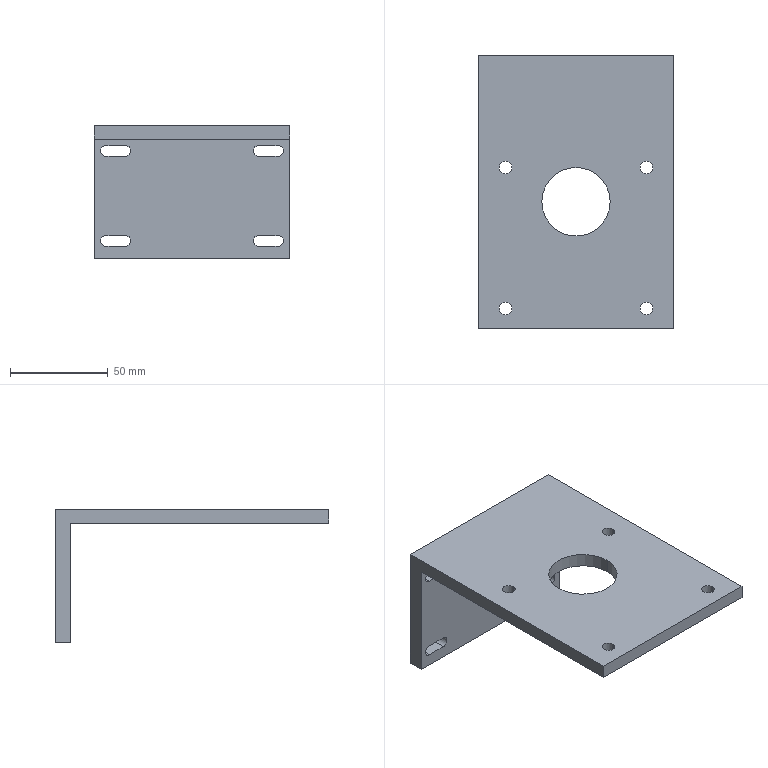Component | SolidWorks | --MA18S2004111xlMotorMountOutline2-1 | 1 solid | 34 faces | box 100 x 140 x 68 mm | volume 136616 mm3 | cylinder 18 | plane 16 | commonest cylinder face diameters 6.5 x8 5.5 x8 35 x2
STEP:
#1=CARTESIAN_POINT('',(11.226,-4.953,2.402));
#2=VERTEX_POINT('',#1);
#3=CARTESIAN_POINT('',(10.97,-4.953,2.402));
#4=VERTEX_POINT('',#3);
#5=CARTESIAN_POINT('',(11.098,-4.953,2.402));
#6=DIRECTION('',(0.,-0.,1.));
#7=DIRECTION('',(0.,-1.,0.));
#8=AXIS2_PLACEMENT_3D('',#5,#6,#7);
#9=CIRCLE('',#8,0.128);
#10=EDGE_CURVE('',#2,#4,#9,.T.);
#11=ORIENTED_EDGE('',*,*,#10,.F.);
#12=CARTESIAN_POINT('',(11.226,-4.953,2.677));
#13=VERTEX_POINT('',#12);
#14=CARTESIAN_POINT('',(11.226,-4.953,2.677));
#15=DIRECTION('',(0.,0.,1.));
#16=VECTOR('',#15,39.37);
#17=LINE('',#14,#16);
#18=EDGE_CURVE('',#2,#13,#17,.T.);
#19=ORIENTED_EDGE('',*,*,#18,.T.);
#20=CARTESIAN_POINT('',(10.97,-4.953,2.677));
#21=VERTEX_POINT('',#20);
#22=CARTESIAN_POINT('',(11.098,-4.953,2.677));
#23=DIRECTION('',(0.,0.,1.));
#24=DIRECTION('',(-1.,0.,0.));
#25=AXIS2_PLACEMENT_3D('',#22,#23,#24);
#26=CIRCLE('',#25,0.128);
#27=EDGE_CURVE('',#13,#21,#26,.T.);
#28=ORIENTED_EDGE('',*,*,#27,.T.);
#29=CARTESIAN_POINT('',(10.97,-4.953,2.677));
#30=DIRECTION('',(0.,0.,1.));
#31=VECTOR('',#30,39.37);
#32=LINE('',#29,#31);
#33=EDGE_CURVE('',#4,#21,#32,.T.);
#34=ORIENTED_EDGE('',*,*,#33,.F.);
#35=EDGE_LOOP('',(#11,#19,#28,#34));
#36=FACE_OUTER_BOUND('',#35,.T.);
#37=CARTESIAN_POINT('',(11.098,-4.953,2.677));
#38=DIRECTION('',(0.,0.,1.));
#39=DIRECTION('',(-1.,0.,0.));
#40=AXIS2_PLACEMENT_3D('',#37,#38,#39);
#41=CYLINDRICAL_SURFACE('',#40,0.128);
#42=ADVANCED_FACE('',(#36),#41,.F.);
#43=CARTESIAN_POINT('',(8.391,-4.953,2.402));
#44=VERTEX_POINT('',#43);
#45=CARTESIAN_POINT('',(8.135,-4.953,2.402));
#46=VERTEX_POINT('',#45);
#47=CARTESIAN_POINT('',(8.263,-4.953,2.402));
#48=DIRECTION('',(0.,-0.,1.));
#49=DIRECTION('',(0.,-1.,0.));
#50=AXIS2_PLACEMENT_3D('',#47,#48,#49);
#51=CIRCLE('',#50,0.128);
#52=EDGE_CURVE('',#44,#46,#51,.T.);
#53=ORIENTED_EDGE('',*,*,#52,.F.);
#54=CARTESIAN_POINT('',(8.391,-4.953,2.677));
#55=VERTEX_POINT('',#54);
#56=CARTESIAN_POINT('',(8.391,-4.953,2.677));
#57=DIRECTION('',(0.,0.,1.));
#58=VECTOR('',#57,39.37);
#59=LINE('',#56,#58);
#60=EDGE_CURVE('',#44,#55,#59,.T.);
#61=ORIENTED_EDGE('',*,*,#60,.T.);
#62=CARTESIAN_POINT('',(8.135,-4.953,2.677));
#63=VERTEX_POINT('',#62);
#64=CARTESIAN_POINT('',(8.263,-4.953,2.677));
#65=DIRECTION('',(0.,0.,1.));
#66=DIRECTION('',(-1.,0.,0.));
#67=AXIS2_PLACEMENT_3D('',#64,#65,#66);
#68=CIRCLE('',#67,0.128);
#69=EDGE_CURVE('',#55,#63,#68,.T.);
#70=ORIENTED_EDGE('',*,*,#69,.T.);
#71=CARTESIAN_POINT('',(8.135,-4.953,2.677));
#72=DIRECTION('',(0.,0.,1.));
#73=VECTOR('',#72,39.37);
#74=LINE('',#71,#73);
#75=EDGE_CURVE('',#46,#63,#74,.T.);
#76=ORIENTED_EDGE('',*,*,#75,.F.);
#77=EDGE_LOOP('',(#53,#61,#70,#76));
#78=FACE_OUTER_BOUND('',#77,.T.);
#79=CARTESIAN_POINT('',(8.263,-4.953,2.677));
#80=DIRECTION('',(0.,0.,1.));
#81=DIRECTION('',(-1.,0.,0.));
#82=AXIS2_PLACEMENT_3D('',#79,#80,#81);
#83=CYLINDRICAL_SURFACE('',#82,0.128);
#84=ADVANCED_FACE('',(#78),#83,.F.);
#85=CARTESIAN_POINT('',(11.226,-2.118,2.402));
#86=VERTEX_POINT('',#85);
#87=CARTESIAN_POINT('',(10.97,-2.118,2.402));
#88=VERTEX_POINT('',#87);
#89=CARTESIAN_POINT('',(11.098,-2.118,2.402));
#90=DIRECTION('',(0.,-0.,1.));
#91=DIRECTION('',(0.,-1.,0.));
#92=AXIS2_PLACEMENT_3D('',#89,#90,#91);
#93=CIRCLE('',#92,0.128);
#94=EDGE_CURVE('',#86,#88,#93,.T.);
#95=ORIENTED_EDGE('',*,*,#94,.F.);
#96=CARTESIAN_POINT('',(11.226,-2.118,2.677));
#97=VERTEX_POINT('',#96);
#98=CARTESIAN_POINT('',(11.226,-2.118,2.677));
#99=DIRECTION('',(0.,0.,1.));
#100=VECTOR('',#99,39.37);
#101=LINE('',#98,#100);
#102=EDGE_CURVE('',#86,#97,#101,.T.);
#103=ORIENTED_EDGE('',*,*,#102,.T.);
#104=CARTESIAN_POINT('',(10.97,-2.118,2.677));
#105=VERTEX_POINT('',#104);
#106=CARTESIAN_POINT('',(11.098,-2.118,2.677));
#107=DIRECTION('',(0.,0.,1.));
#108=DIRECTION('',(-1.,0.,0.));
#109=AXIS2_PLACEMENT_3D('',#106,#107,#108);
#110=CIRCLE('',#109,0.128);
#111=EDGE_CURVE('',#97,#105,#110,.T.);
#112=ORIENTED_EDGE('',*,*,#111,.T.);
#113=CARTESIAN_POINT('',(10.97,-2.118,2.677));
#114=DIRECTION('',(0.,0.,1.));
#115=VECTOR('',#114,39.37);
#116=LINE('',#113,#115);
#117=EDGE_CURVE('',#88,#105,#116,.T.);
#118=ORIENTED_EDGE('',*,*,#117,.F.);
#119=EDGE_LOOP('',(#95,#103,#112,#118));
#120=FACE_OUTER_BOUND('',#119,.T.);
#121=CARTESIAN_POINT('',(11.098,-2.118,2.677));
#122=DIRECTION('',(0.,0.,1.));
#123=DIRECTION('',(-1.,0.,0.));
#124=AXIS2_PLACEMENT_3D('',#121,#122,#123);
#125=CYLINDRICAL_SURFACE('',#124,0.128);
#126=ADVANCED_FACE('',(#120),#125,.F.);
#127=CARTESIAN_POINT('',(8.391,-2.118,2.402));
#128=VERTEX_POINT('',#127);
#129=CARTESIAN_POINT('',(8.135,-2.118,2.402));
#130=VERTEX_POINT('',#129);
#131=CARTESIAN_POINT('',(8.263,-2.118,2.402));
#132=DIRECTION('',(0.,-0.,1.));
#133=DIRECTION('',(0.,-1.,0.));
#134=AXIS2_PLACEMENT_3D('',#131,#132,#133);
#135=CIRCLE('',#134,0.128);
#136=EDGE_CURVE('',#128,#130,#135,.T.);
#137=ORIENTED_EDGE('',*,*,#136,.F.);
#138=CARTESIAN_POINT('',(8.391,-2.118,2.677));
#139=VERTEX_POINT('',#138);
#140=CARTESIAN_POINT('',(8.391,-2.118,2.677));
#141=DIRECTION('',(0.,0.,1.));
#142=VECTOR('',#141,39.37);
#143=LINE('',#140,#142);
#144=EDGE_CURVE('',#128,#139,#143,.T.);
#145=ORIENTED_EDGE('',*,*,#144,.T.);
#146=CARTESIAN_POINT('',(8.135,-2.118,2.677));
#147=VERTEX_POINT('',#146);
#148=CARTESIAN_POINT('',(8.263,-2.118,2.677));
#149=DIRECTION('',(0.,0.,1.));
#150=DIRECTION('',(-1.,0.,0.));
#151=AXIS2_PLACEMENT_3D('',#148,#149,#150);
#152=CIRCLE('',#151,0.128);
#153=EDGE_CURVE('',#139,#147,#152,.T.);
#154=ORIENTED_EDGE('',*,*,#153,.T.);
#155=CARTESIAN_POINT('',(8.135,-2.118,2.677));
#156=DIRECTION('',(0.,0.,1.));
#157=VECTOR('',#156,39.37);
#158=LINE('',#155,#157);
#159=EDGE_CURVE('',#130,#147,#158,.T.);
#160=ORIENTED_EDGE('',*,*,#159,.F.);
#161=EDGE_LOOP('',(#137,#145,#154,#160));
#162=FACE_OUTER_BOUND('',#161,.T.);
#163=CARTESIAN_POINT('',(8.263,-2.118,2.677));
#164=DIRECTION('',(0.,0.,1.));
#165=DIRECTION('',(-1.,0.,0.));
#166=AXIS2_PLACEMENT_3D('',#163,#164,#165);
#167=CYLINDRICAL_SURFACE('',#166,0.128);
#168=ADVANCED_FACE('',(#162),#167,.F.);
#169=CARTESIAN_POINT('',(10.369,-2.807,2.402));
#170=VERTEX_POINT('',#169);
#171=CARTESIAN_POINT('',(8.992,-2.807,2.402));
#172=VERTEX_POINT('',#171);
#173=CARTESIAN_POINT('',(9.681,-2.807,2.402));
#174=DIRECTION('',(0.,-0.,1.));
#175=DIRECTION('',(0.,-1.,0.));
#176=AXIS2_PLACEMENT_3D('',#173,#174,#175);
#177=CIRCLE('',#176,0.689);
#178=EDGE_CURVE('',#170,#172,#177,.T.);
#179=ORIENTED_EDGE('',*,*,#178,.F.);
#180=CARTESIAN_POINT('',(10.369,-2.807,2.677));
#181=VERTEX_POINT('',#180);
#182=CARTESIAN_POINT('',(10.369,-2.807,0.));
#183=DIRECTION('',(0.,0.,1.));
#184=VECTOR('',#183,39.37);
#185=LINE('',#182,#184);
#186=EDGE_CURVE('',#170,#181,#185,.T.);
#187=ORIENTED_EDGE('',*,*,#186,.T.);
#188=CARTESIAN_POINT('',(8.992,-2.807,2.677));
#189=VERTEX_POINT('',#188);
#190=CARTESIAN_POINT('',(9.681,-2.807,2.677));
#191=DIRECTION('',(0.,0.,1.));
#192=DIRECTION('',(-1.,0.,0.));
#193=AXIS2_PLACEMENT_3D('',#190,#191,#192);
#194=CIRCLE('',#193,0.689);
#195=EDGE_CURVE('',#181,#189,#194,.T.);
#196=ORIENTED_EDGE('',*,*,#195,.T.);
#197=CARTESIAN_POINT('',(8.992,-2.807,0.));
#198=DIRECTION('',(0.,0.,1.));
#199=VECTOR('',#198,39.37);
#200=LINE('',#197,#199);
#201=EDGE_CURVE('',#172,#189,#200,.T.);
#202=ORIENTED_EDGE('',*,*,#201,.F.);
#203=EDGE_LOOP('',(#179,#187,#196,#202));
#204=FACE_OUTER_BOUND('',#203,.T.);
#205=CARTESIAN_POINT('',(9.681,-2.807,0.));
#206=DIRECTION('',(0.,0.,1.));
#207=DIRECTION('',(-1.,0.,0.));
#208=AXIS2_PLACEMENT_3D('',#205,#206,#207);
#209=CYLINDRICAL_SURFACE('',#208,0.689);
#210=ADVANCED_FACE('',(#204),#209,.F.);
#211=CARTESIAN_POINT('',(7.948,0.1456,2.057));
#212=VERTEX_POINT('',#211);
#213=CARTESIAN_POINT('',(8.342,0.1456,2.057));
#214=VERTEX_POINT('',#213);
#215=CARTESIAN_POINT('',(8.342,0.1456,2.057));
#216=DIRECTION('',(1.,0.,0.));
#217=VECTOR('',#216,39.37);
#218=LINE('',#215,#217);
#219=EDGE_CURVE('',#212,#214,#218,.T.);
#220=ORIENTED_EDGE('',*,*,#219,.T.);
#221=CARTESIAN_POINT('',(8.342,0.1456,2.274));
#222=VERTEX_POINT('',#221);
#223=CARTESIAN_POINT('',(8.342,0.1456,2.165));
#224=DIRECTION('',(0.,-1.,-0.));
#225=DIRECTION('',(0.,0.,-1.));
#226=AXIS2_PLACEMENT_3D('',#223,#224,#225);
#227=CIRCLE('',#226,0.1083);
#228=EDGE_CURVE('',#214,#222,#227,.T.);
#229=ORIENTED_EDGE('',*,*,#228,.T.);
#230=CARTESIAN_POINT('',(7.948,0.1456,2.274));
#231=VERTEX_POINT('',#230);
#232=CARTESIAN_POINT('',(8.342,0.1456,2.274));
#233=DIRECTION('',(-1.,0.,0.));
#234=VECTOR('',#233,39.37);
#235=LINE('',#232,#234);
#236=EDGE_CURVE('',#222,#231,#235,.T.);
#237=ORIENTED_EDGE('',*,*,#236,.T.);
#238=CARTESIAN_POINT('',(7.948,0.1456,2.165));
#239=DIRECTION('',(0.,-1.,-0.));
#240=DIRECTION('',(0.,0.,-1.));
#241=AXIS2_PLACEMENT_3D('',#238,#239,#240);
#242=CIRCLE('',#241,0.1083);
#243=EDGE_CURVE('',#231,#212,#242,.T.);
#244=ORIENTED_EDGE('',*,*,#243,.T.);
#245=EDGE_LOOP('',(#220,#229,#237,#244));
#246=FACE_BOUND('',#245,.T.);
#247=CARTESIAN_POINT('',(11.019,0.1456,2.057));
#248=VERTEX_POINT('',#247);
#249=CARTESIAN_POINT('',(11.413,0.1456,2.057));
#250=VERTEX_POINT('',#249);
#251=CARTESIAN_POINT('',(11.413,0.1456,2.057));
#252=DIRECTION('',(1.,0.,0.));
#253=VECTOR('',#252,39.37);
#254=LINE('',#251,#253);
#255=EDGE_CURVE('',#248,#250,#254,.T.);
#256=ORIENTED_EDGE('',*,*,#255,.T.);
#257=CARTESIAN_POINT('',(11.413,0.1456,2.274));
#258=VERTEX_POINT('',#257);
#259=CARTESIAN_POINT('',(11.413,0.1456,2.165));
#260=DIRECTION('',(0.,-1.,-0.));
#261=DIRECTION('',(0.,0.,-1.));
#262=AXIS2_PLACEMENT_3D('',#259,#260,#261);
#263=CIRCLE('',#262,0.1083);
#264=EDGE_CURVE('',#250,#258,#263,.T.);
#265=ORIENTED_EDGE('',*,*,#264,.T.);
#266=CARTESIAN_POINT('',(11.019,0.1456,2.274));
#267=VERTEX_POINT('',#266);
#268=CARTESIAN_POINT('',(11.413,0.1456,2.274));
#269=DIRECTION('',(-1.,0.,0.));
#270=VECTOR('',#269,39.37);
#271=LINE('',#268,#270);
#272=EDGE_CURVE('',#258,#267,#271,.T.);
#273=ORIENTED_EDGE('',*,*,#272,.T.);
#274=CARTESIAN_POINT('',(11.019,0.1456,2.165));
#275=DIRECTION('',(0.,-1.,-0.));
#276=DIRECTION('',(0.,0.,-1.));
#277=AXIS2_PLACEMENT_3D('',#274,#275,#276);
#278=CIRCLE('',#277,0.1083);
#279=EDGE_CURVE('',#267,#248,#278,.T.);
#280=ORIENTED_EDGE('',*,*,#279,.T.);
#281=EDGE_LOOP('',(#256,#265,#273,#280));
#282=FACE_BOUND('',#281,.T.);
#283=CARTESIAN_POINT('',(7.948,0.1456,0.2461));
#284=VERTEX_POINT('',#283);
#285=CARTESIAN_POINT('',(8.342,0.1456,0.2461));
#286=VERTEX_POINT('',#285);
#287=CARTESIAN_POINT('',(8.342,0.1456,0.2461));
#288=DIRECTION('',(1.,0.,0.));
#289=VECTOR('',#288,39.37);
#290=LINE('',#287,#289);
#291=EDGE_CURVE('',#284,#286,#290,.T.);
#292=ORIENTED_EDGE('',*,*,#291,.T.);
#293=CARTESIAN_POINT('',(8.342,0.1456,0.4626));
#294=VERTEX_POINT('',#293);
#295=CARTESIAN_POINT('',(8.342,0.1456,0.3543));
#296=DIRECTION('',(0.,-1.,-0.));
#297=DIRECTION('',(0.,0.,-1.));
#298=AXIS2_PLACEMENT_3D('',#295,#296,#297);
#299=CIRCLE('',#298,0.1083);
#300=EDGE_CURVE('',#286,#294,#299,.T.);
#301=ORIENTED_EDGE('',*,*,#300,.T.);
#302=CARTESIAN_POINT('',(7.948,0.1456,0.4626));
#303=VERTEX_POINT('',#302);
#304=CARTESIAN_POINT('',(8.342,0.1456,0.4626));
#305=DIRECTION('',(-1.,0.,0.));
#306=VECTOR('',#305,39.37);
#307=LINE('',#304,#306);
#308=EDGE_CURVE('',#294,#303,#307,.T.);
#309=ORIENTED_EDGE('',*,*,#308,.T.);
#310=CARTESIAN_POINT('',(7.948,0.1456,0.3543));
#311=DIRECTION('',(0.,-1.,-0.));
#312=DIRECTION('',(0.,0.,-1.));
#313=AXIS2_PLACEMENT_3D('',#310,#311,#312);
#314=CIRCLE('',#313,0.1083);
#315=EDGE_CURVE('',#303,#284,#314,.T.);
#316=ORIENTED_EDGE('',*,*,#315,.T.);
#317=EDGE_LOOP('',(#292,#301,#309,#316));
#318=FACE_BOUND('',#317,.T.);
#319=CARTESIAN_POINT('',(11.019,0.1456,0.2461));
#320=VERTEX_POINT('',#319);
#321=CARTESIAN_POINT('',(11.413,0.1456,0.2461));
#322=VERTEX_POINT('',#321);
#323=CARTESIAN_POINT('',(11.413,0.1456,0.2461));
#324=DIRECTION('',(1.,0.,0.));
#325=VECTOR('',#324,39.37);
#326=LINE('',#323,#325);
#327=EDGE_CURVE('',#320,#322,#326,.T.);
#328=ORIENTED_EDGE('',*,*,#327,.T.);
#329=CARTESIAN_POINT('',(11.413,0.1456,0.4626));
#330=VERTEX_POINT('',#329);
#331=CARTESIAN_POINT('',(11.413,0.1456,0.3543));
#332=DIRECTION('',(0.,-1.,-0.));
#333=DIRECTION('',(0.,0.,-1.));
#334=AXIS2_PLACEMENT_3D('',#331,#332,#333);
#335=CIRCLE('',#334,0.1083);
#336=EDGE_CURVE('',#322,#330,#335,.T.);
#337=ORIENTED_EDGE('',*,*,#336,.T.);
#338=CARTESIAN_POINT('',(11.019,0.1456,0.4626));
#339=VERTEX_POINT('',#338);
#340=CARTESIAN_POINT('',(11.413,0.1456,0.4626));
#341=DIRECTION('',(-1.,0.,0.));
#342=VECTOR('',#341,39.37);
#343=LINE('',#340,#342);
#344=EDGE_CURVE('',#330,#339,#343,.T.);
#345=ORIENTED_EDGE('',*,*,#344,.T.);
#346=CARTESIAN_POINT('',(11.019,0.1456,0.3543));
#347=DIRECTION('',(0.,-1.,-0.));
#348=DIRECTION('',(0.,0.,-1.));
#349=AXIS2_PLACEMENT_3D('',#346,#347,#348);
#350=CIRCLE('',#349,0.1083);
#351=EDGE_CURVE('',#339,#320,#350,.T.);
#352=ORIENTED_EDGE('',*,*,#351,.T.);
#353=EDGE_LOOP('',(#328,#337,#345,#352));
#354=FACE_BOUND('',#353,.T.);
#355=CARTESIAN_POINT('',(7.712,0.1456,0.));
#356=VERTEX_POINT('',#355);
#357=CARTESIAN_POINT('',(7.712,0.1456,2.677));
#358=VERTEX_POINT('',#357);
#359=CARTESIAN_POINT('',(7.712,0.1456,2.677));
#360=DIRECTION('',(0.,0.,1.));
#361=VECTOR('',#360,39.37);
#362=LINE('',#359,#361);
#363=EDGE_CURVE('',#356,#358,#362,.T.);
#364=ORIENTED_EDGE('',*,*,#363,.T.);
#365=CARTESIAN_POINT('',(11.649,0.1456,2.677));
#366=VERTEX_POINT('',#365);
#367=CARTESIAN_POINT('',(11.649,0.1456,2.677));
#368=DIRECTION('',(-1.,0.,0.));
#369=VECTOR('',#368,39.37);
#370=LINE('',#367,#369);
#371=EDGE_CURVE('',#366,#358,#370,.T.);
#372=ORIENTED_EDGE('',*,*,#371,.F.);
#373=CARTESIAN_POINT('',(11.649,0.1456,0.));
#374=VERTEX_POINT('',#373);
#375=CARTESIAN_POINT('',(11.649,0.1456,2.677));
#376=DIRECTION('',(0.,0.,1.));
#377=VECTOR('',#376,39.37);
#378=LINE('',#375,#377);
#379=EDGE_CURVE('',#374,#366,#378,.T.);
#380=ORIENTED_EDGE('',*,*,#379,.F.);
#381=CARTESIAN_POINT('',(11.649,0.1456,0.));
#382=DIRECTION('',(-1.,0.,0.));
#383=VECTOR('',#382,39.37);
#384=LINE('',#381,#383);
#385=EDGE_CURVE('',#374,#356,#384,.T.);
#386=ORIENTED_EDGE('',*,*,#385,.T.);
#387=EDGE_LOOP('',(#364,#372,#380,#386));
#388=FACE_OUTER_BOUND('',#387,.T.);
#389=CARTESIAN_POINT('',(11.649,0.1456,2.677));
#390=DIRECTION('',(0.,-1.,0.));
#391=DIRECTION('',(-1.,0.,0.));
#392=AXIS2_PLACEMENT_3D('',#389,#390,#391);
#393=PLANE('',#392);
#394=ADVANCED_FACE('',(#246,#282,#318,#354,#388),#393,.F.);
#395=CARTESIAN_POINT('',(11.098,-4.953,2.677));
#396=DIRECTION('',(0.,0.,1.));
#397=DIRECTION('',(-1.,0.,0.));
#398=AXIS2_PLACEMENT_3D('',#395,#396,#397);
#399=CIRCLE('',#398,0.128);
#400=EDGE_CURVE('',#21,#13,#399,.T.);
#401=ORIENTED_EDGE('',*,*,#400,.F.);
#402=ORIENTED_EDGE('',*,*,#27,.F.);
#403=EDGE_LOOP('',(#401,#402));
#404=FACE_BOUND('',#403,.T.);
#405=CARTESIAN_POINT('',(8.263,-4.953,2.677));
#406=DIRECTION('',(0.,0.,1.));
#407=DIRECTION('',(-1.,0.,0.));
#408=AXIS2_PLACEMENT_3D('',#405,#406,#407);
#409=CIRCLE('',#408,0.128);
#410=EDGE_CURVE('',#63,#55,#409,.T.);
#411=ORIENTED_EDGE('',*,*,#410,.F.);
#412=ORIENTED_EDGE('',*,*,#69,.F.);
#413=EDGE_LOOP('',(#411,#412));
#414=FACE_BOUND('',#413,.T.);
#415=CARTESIAN_POINT('',(11.098,-2.118,2.677));
#416=DIRECTION('',(0.,0.,1.));
#417=DIRECTION('',(-1.,0.,0.));
#418=AXIS2_PLACEMENT_3D('',#415,#416,#417);
#419=CIRCLE('',#418,0.128);
#420=EDGE_CURVE('',#105,#97,#419,.T.);
#421=ORIENTED_EDGE('',*,*,#420,.F.);
#422=ORIENTED_EDGE('',*,*,#111,.F.);
#423=EDGE_LOOP('',(#421,#422));
#424=FACE_BOUND('',#423,.T.);
#425=CARTESIAN_POINT('',(8.263,-2.118,2.677));
#426=DIRECTION('',(0.,0.,1.));
#427=DIRECTION('',(-1.,0.,0.));
#428=AXIS2_PLACEMENT_3D('',#425,#426,#427);
#429=CIRCLE('',#428,0.128);
#430=EDGE_CURVE('',#147,#139,#429,.T.);
#431=ORIENTED_EDGE('',*,*,#430,.F.);
#432=ORIENTED_EDGE('',*,*,#153,.F.);
#433=EDGE_LOOP('',(#431,#432));
#434=FACE_BOUND('',#433,.T.);
#435=CARTESIAN_POINT('',(9.681,-2.807,2.677));
#436=DIRECTION('',(0.,0.,1.));
#437=DIRECTION('',(-1.,0.,0.));
#438=AXIS2_PLACEMENT_3D('',#435,#436,#437);
#439=CIRCLE('',#438,0.689);
#440=EDGE_CURVE('',#189,#181,#439,.T.);
#441=ORIENTED_EDGE('',*,*,#440,.F.);
#442=ORIENTED_EDGE('',*,*,#195,.F.);
#443=EDGE_LOOP('',(#441,#442));
#444=FACE_BOUND('',#443,.T.);
#445=CARTESIAN_POINT('',(7.712,-5.366,2.677));
#446=VERTEX_POINT('',#445);
#447=CARTESIAN_POINT('',(7.712,0.1456,2.677));
#448=DIRECTION('',(0.,-1.,0.));
#449=VECTOR('',#448,39.37);
#450=LINE('',#447,#449);
#451=EDGE_CURVE('',#358,#446,#450,.T.);
#452=ORIENTED_EDGE('',*,*,#451,.T.);
#453=CARTESIAN_POINT('',(11.649,-5.366,2.677));
#454=VERTEX_POINT('',#453);
#455=CARTESIAN_POINT('',(11.649,-5.366,2.677));
#456=DIRECTION('',(-1.,0.,0.));
#457=VECTOR('',#456,39.37);
#458=LINE('',#455,#457);
#459=EDGE_CURVE('',#454,#446,#458,.T.);
#460=ORIENTED_EDGE('',*,*,#459,.F.);
#461=CARTESIAN_POINT('',(11.649,0.1456,2.677));
#462=DIRECTION('',(0.,-1.,0.));
#463=VECTOR('',#462,39.37);
#464=LINE('',#461,#463);
#465=EDGE_CURVE('',#366,#454,#464,.T.);
#466=ORIENTED_EDGE('',*,*,#465,.F.);
#467=ORIENTED_EDGE('',*,*,#371,.T.);
#468=EDGE_LOOP('',(#452,#460,#466,#467));
#469=FACE_OUTER_BOUND('',#468,.T.);
#470=CARTESIAN_POINT('',(11.649,0.1456,2.677));
#471=DIRECTION('',(0.,0.,-1.));
#472=DIRECTION('',(1.,0.,0.));
#473=AXIS2_PLACEMENT_3D('',#470,#471,#472);
#474=PLANE('',#473);
#475=ADVANCED_FACE('',(#404,#414,#424,#434,#444,#469),#474,.F.);
#476=CARTESIAN_POINT('',(7.712,-5.366,2.402));
#477=VERTEX_POINT('',#476);
#478=CARTESIAN_POINT('',(7.712,-5.366,2.677));
#479=DIRECTION('',(0.,0.,-1.));
#480=VECTOR('',#479,39.37);
#481=LINE('',#478,#480);
#482=EDGE_CURVE('',#446,#477,#481,.T.);
#483=ORIENTED_EDGE('',*,*,#482,.T.);
#484=CARTESIAN_POINT('',(11.649,-5.366,2.402));
#485=VERTEX_POINT('',#484);
#486=CARTESIAN_POINT('',(11.649,-5.366,2.402));
#487=DIRECTION('',(-1.,0.,0.));
#488=VECTOR('',#487,39.37);
#489=LINE('',#486,#488);
#490=EDGE_CURVE('',#485,#477,#489,.T.);
#491=ORIENTED_EDGE('',*,*,#490,.F.);
#492=CARTESIAN_POINT('',(11.649,-5.366,2.677));
#493=DIRECTION('',(0.,0.,-1.));
#494=VECTOR('',#493,39.37);
#495=LINE('',#492,#494);
#496=EDGE_CURVE('',#454,#485,#495,.T.);
#497=ORIENTED_EDGE('',*,*,#496,.F.);
#498=ORIENTED_EDGE('',*,*,#459,.T.);
#499=EDGE_LOOP('',(#483,#491,#497,#498));
#500=FACE_OUTER_BOUND('',#499,.T.);
#501=CARTESIAN_POINT('',(11.649,-5.366,2.677));
#502=DIRECTION('',(0.,1.,0.));
#503=DIRECTION('',(1.,0.,0.));
#504=AXIS2_PLACEMENT_3D('',#501,#502,#503);
#505=PLANE('',#504);
#506=ADVANCED_FACE('',(#500),#505,.F.);
#507=CARTESIAN_POINT('',(11.098,-4.953,2.402));
#508=DIRECTION('',(0.,-0.,1.));
#509=DIRECTION('',(0.,-1.,0.));
#510=AXIS2_PLACEMENT_3D('',#507,#508,#509);
#511=CIRCLE('',#510,0.128);
#512=EDGE_CURVE('',#4,#2,#511,.T.);
#513=ORIENTED_EDGE('',*,*,#512,.T.);
#514=ORIENTED_EDGE('',*,*,#10,.T.);
#515=EDGE_LOOP('',(#513,#514));
#516=FACE_BOUND('',#515,.T.);
#517=CARTESIAN_POINT('',(8.263,-4.953,2.402));
#518=DIRECTION('',(0.,-0.,1.));
#519=DIRECTION('',(0.,-1.,0.));
#520=AXIS2_PLACEMENT_3D('',#517,#518,#519);
#521=CIRCLE('',#520,0.128);
#522=EDGE_CURVE('',#46,#44,#521,.T.);
#523=ORIENTED_EDGE('',*,*,#522,.T.);
#524=ORIENTED_EDGE('',*,*,#52,.T.);
#525=EDGE_LOOP('',(#523,#524));
#526=FACE_BOUND('',#525,.T.);
#527=CARTESIAN_POINT('',(11.098,-2.118,2.402));
#528=DIRECTION('',(0.,-0.,1.));
#529=DIRECTION('',(0.,-1.,0.));
#530=AXIS2_PLACEMENT_3D('',#527,#528,#529);
#531=CIRCLE('',#530,0.128);
#532=EDGE_CURVE('',#88,#86,#531,.T.);
#533=ORIENTED_EDGE('',*,*,#532,.T.);
#534=ORIENTED_EDGE('',*,*,#94,.T.);
#535=EDGE_LOOP('',(#533,#534));
#536=FACE_BOUND('',#535,.T.);
#537=CARTESIAN_POINT('',(8.263,-2.118,2.402));
#538=DIRECTION('',(0.,-0.,1.));
#539=DIRECTION('',(0.,-1.,0.));
#540=AXIS2_PLACEMENT_3D('',#537,#538,#539);
#541=CIRCLE('',#540,0.128);
#542=EDGE_CURVE('',#130,#128,#541,.T.);
#543=ORIENTED_EDGE('',*,*,#542,.T.);
#544=ORIENTED_EDGE('',*,*,#136,.T.);
#545=EDGE_LOOP('',(#543,#544));
#546=FACE_BOUND('',#545,.T.);
#547=CARTESIAN_POINT('',(9.681,-2.807,2.402));
#548=DIRECTION('',(0.,-0.,1.));
#549=DIRECTION('',(0.,-1.,0.));
#550=AXIS2_PLACEMENT_3D('',#547,#548,#549);
#551=CIRCLE('',#550,0.689);
#552=EDGE_CURVE('',#172,#170,#551,.T.);
#553=ORIENTED_EDGE('',*,*,#552,.T.);
#554=ORIENTED_EDGE('',*,*,#178,.T.);
#555=EDGE_LOOP('',(#553,#554));
#556=FACE_BOUND('',#555,.T.);
#557=CARTESIAN_POINT('',(7.712,-0.1693,2.402));
#558=VERTEX_POINT('',#557);
#559=CARTESIAN_POINT('',(7.712,-5.366,2.402));
#560=DIRECTION('',(0.,1.,0.));
#561=VECTOR('',#560,39.37);
#562=LINE('',#559,#561);
#563=EDGE_CURVE('',#477,#558,#562,.T.);
#564=ORIENTED_EDGE('',*,*,#563,.T.);
#565=CARTESIAN_POINT('',(11.649,-0.1693,2.402));
#566=VERTEX_POINT('',#565);
#567=CARTESIAN_POINT('',(11.649,-0.1693,2.402));
#568=DIRECTION('',(-1.,0.,0.));
#569=VECTOR('',#568,39.37);
#570=LINE('',#567,#569);
#571=EDGE_CURVE('',#566,#558,#570,.T.);
#572=ORIENTED_EDGE('',*,*,#571,.F.);
#573=CARTESIAN_POINT('',(11.649,-5.366,2.402));
#574=DIRECTION('',(0.,1.,0.));
#575=VECTOR('',#574,39.37);
#576=LINE('',#573,#575);
#577=EDGE_CURVE('',#485,#566,#576,.T.);
#578=ORIENTED_EDGE('',*,*,#577,.F.);
#579=ORIENTED_EDGE('',*,*,#490,.T.);
#580=EDGE_LOOP('',(#564,#572,#578,#579));
#581=FACE_OUTER_BOUND('',#580,.T.);
#582=CARTESIAN_POINT('',(11.649,-5.366,2.402));
#583=DIRECTION('',(0.,-0.,1.));
#584=DIRECTION('',(0.,-1.,-0.));
#585=AXIS2_PLACEMENT_3D('',#582,#583,#584);
#586=PLANE('',#585);
#587=ADVANCED_FACE('',(#516,#526,#536,#546,#556,#581),#586,.F.);
#588=CARTESIAN_POINT('',(8.342,-0.1693,2.274));
#589=VERTEX_POINT('',#588);
#590=CARTESIAN_POINT('',(7.948,-0.1693,2.274));
#591=VERTEX_POINT('',#590);
#592=CARTESIAN_POINT('',(8.342,-0.1693,2.274));
#593=DIRECTION('',(-1.,0.,0.));
#594=VECTOR('',#593,39.37);
#595=LINE('',#592,#594);
#596=EDGE_CURVE('',#589,#591,#595,.T.);
#597=ORIENTED_EDGE('',*,*,#596,.F.);
#598=CARTESIAN_POINT('',(8.342,-0.1693,2.057));
#599=VERTEX_POINT('',#598);
#600=CARTESIAN_POINT('',(8.342,-0.1693,2.165));
#601=DIRECTION('',(0.,-1.,-0.));
#602=DIRECTION('',(0.,0.,-1.));
#603=AXIS2_PLACEMENT_3D('',#600,#601,#602);
#604=CIRCLE('',#603,0.1083);
#605=EDGE_CURVE('',#599,#589,#604,.T.);
#606=ORIENTED_EDGE('',*,*,#605,.F.);
#607=CARTESIAN_POINT('',(7.948,-0.1693,2.057));
#608=VERTEX_POINT('',#607);
#609=CARTESIAN_POINT('',(8.342,-0.1693,2.057));
#610=DIRECTION('',(1.,0.,0.));
#611=VECTOR('',#610,39.37);
#612=LINE('',#609,#611);
#613=EDGE_CURVE('',#608,#599,#612,.T.);
#614=ORIENTED_EDGE('',*,*,#613,.F.);
#615=CARTESIAN_POINT('',(7.948,-0.1693,2.165));
#616=DIRECTION('',(0.,-1.,-0.));
#617=DIRECTION('',(0.,0.,-1.));
#618=AXIS2_PLACEMENT_3D('',#615,#616,#617);
#619=CIRCLE('',#618,0.1083);
#620=EDGE_CURVE('',#591,#608,#619,.T.);
#621=ORIENTED_EDGE('',*,*,#620,.F.);
#622=EDGE_LOOP('',(#597,#606,#614,#621));
#623=FACE_BOUND('',#622,.T.);
#624=CARTESIAN_POINT('',(11.413,-0.1693,2.274));
#625=VERTEX_POINT('',#624);
#626=CARTESIAN_POINT('',(11.019,-0.1693,2.274));
#627=VERTEX_POINT('',#626);
#628=CARTESIAN_POINT('',(11.413,-0.1693,2.274));
#629=DIRECTION('',(-1.,0.,0.));
#630=VECTOR('',#629,39.37);
#631=LINE('',#628,#630);
#632=EDGE_CURVE('',#625,#627,#631,.T.);
#633=ORIENTED_EDGE('',*,*,#632,.F.);
#634=CARTESIAN_POINT('',(11.413,-0.1693,2.057));
#635=VERTEX_POINT('',#634);
#636=CARTESIAN_POINT('',(11.413,-0.1693,2.165));
#637=DIRECTION('',(0.,-1.,-0.));
#638=DIRECTION('',(0.,0.,-1.));
#639=AXIS2_PLACEMENT_3D('',#636,#637,#638);
#640=CIRCLE('',#639,0.1083);
#641=EDGE_CURVE('',#635,#625,#640,.T.);
#642=ORIENTED_EDGE('',*,*,#641,.F.);
#643=CARTESIAN_POINT('',(11.019,-0.1693,2.057));
#644=VERTEX_POINT('',#643);
#645=CARTESIAN_POINT('',(11.413,-0.1693,2.057));
#646=DIRECTION('',(1.,0.,0.));
#647=VECTOR('',#646,39.37);
#648=LINE('',#645,#647);
#649=EDGE_CURVE('',#644,#635,#648,.T.);
#650=ORIENTED_EDGE('',*,*,#649,.F.);
#651=CARTESIAN_POINT('',(11.019,-0.1693,2.165));
#652=DIRECTION('',(0.,-1.,-0.));
#653=DIRECTION('',(0.,0.,-1.));
#654=AXIS2_PLACEMENT_3D('',#651,#652,#653);
#655=CIRCLE('',#654,0.1083);
#656=EDGE_CURVE('',#627,#644,#655,.T.);
#657=ORIENTED_EDGE('',*,*,#656,.F.);
#658=EDGE_LOOP('',(#633,#642,#650,#657));
#659=FACE_BOUND('',#658,.T.);
#660=CARTESIAN_POINT('',(8.342,-0.1693,0.4626));
#661=VERTEX_POINT('',#660);
#662=CARTESIAN_POINT('',(7.948,-0.1693,0.4626));
#663=VERTEX_POINT('',#662);
#664=CARTESIAN_POINT('',(8.342,-0.1693,0.4626));
#665=DIRECTION('',(-1.,0.,0.));
#666=VECTOR('',#665,39.37);
#667=LINE('',#664,#666);
#668=EDGE_CURVE('',#661,#663,#667,.T.);
#669=ORIENTED_EDGE('',*,*,#668,.F.);
#670=CARTESIAN_POINT('',(8.342,-0.1693,0.2461));
#671=VERTEX_POINT('',#670);
#672=CARTESIAN_POINT('',(8.342,-0.1693,0.3543));
#673=DIRECTION('',(0.,-1.,-0.));
#674=DIRECTION('',(0.,0.,-1.));
#675=AXIS2_PLACEMENT_3D('',#672,#673,#674);
#676=CIRCLE('',#675,0.1083);
#677=EDGE_CURVE('',#671,#661,#676,.T.);
#678=ORIENTED_EDGE('',*,*,#677,.F.);
#679=CARTESIAN_POINT('',(7.948,-0.1693,0.2461));
#680=VERTEX_POINT('',#679);
#681=CARTESIAN_POINT('',(8.342,-0.1693,0.2461));
#682=DIRECTION('',(1.,0.,0.));
#683=VECTOR('',#682,39.37);
#684=LINE('',#681,#683);
#685=EDGE_CURVE('',#680,#671,#684,.T.);
#686=ORIENTED_EDGE('',*,*,#685,.F.);
#687=CARTESIAN_POINT('',(7.948,-0.1693,0.3543));
#688=DIRECTION('',(0.,-1.,-0.));
#689=DIRECTION('',(0.,0.,-1.));
#690=AXIS2_PLACEMENT_3D('',#687,#688,#689);
#691=CIRCLE('',#690,0.1083);
#692=EDGE_CURVE('',#663,#680,#691,.T.);
#693=ORIENTED_EDGE('',*,*,#692,.F.);
#694=EDGE_LOOP('',(#669,#678,#686,#693));
#695=FACE_BOUND('',#694,.T.);
#696=CARTESIAN_POINT('',(11.413,-0.1693,0.4626));
#697=VERTEX_POINT('',#696);
#698=CARTESIAN_POINT('',(11.019,-0.1693,0.4626));
#699=VERTEX_POINT('',#698);
#700=CARTESIAN_POINT('',(11.413,-0.1693,0.4626));
#701=DIRECTION('',(-1.,0.,0.));
#702=VECTOR('',#701,39.37);
#703=LINE('',#700,#702);
#704=EDGE_CURVE('',#697,#699,#703,.T.);
#705=ORIENTED_EDGE('',*,*,#704,.F.);
#706=CARTESIAN_POINT('',(11.413,-0.1693,0.2461));
#707=VERTEX_POINT('',#706);
#708=CARTESIAN_POINT('',(11.413,-0.1693,0.3543));
#709=DIRECTION('',(0.,-1.,-0.));
#710=DIRECTION('',(0.,0.,-1.));
#711=AXIS2_PLACEMENT_3D('',#708,#709,#710);
#712=CIRCLE('',#711,0.1083);
#713=EDGE_CURVE('',#707,#697,#712,.T.);
#714=ORIENTED_EDGE('',*,*,#713,.F.);
#715=CARTESIAN_POINT('',(11.019,-0.1693,0.2461));
#716=VERTEX_POINT('',#715);
#717=CARTESIAN_POINT('',(11.413,-0.1693,0.2461));
#718=DIRECTION('',(1.,0.,0.));
#719=VECTOR('',#718,39.37);
#720=LINE('',#717,#719);
#721=EDGE_CURVE('',#716,#707,#720,.T.);
#722=ORIENTED_EDGE('',*,*,#721,.F.);
#723=CARTESIAN_POINT('',(11.019,-0.1693,0.3543));
#724=DIRECTION('',(0.,-1.,-0.));
#725=DIRECTION('',(0.,0.,-1.));
#726=AXIS2_PLACEMENT_3D('',#723,#724,#725);
#727=CIRCLE('',#726,0.1083);
#728=EDGE_CURVE('',#699,#716,#727,.T.);
#729=ORIENTED_EDGE('',*,*,#728,.F.);
#730=EDGE_LOOP('',(#705,#714,#722,#729));
#731=FACE_BOUND('',#730,.T.);
#732=CARTESIAN_POINT('',(7.712,-0.1693,0.));
#733=VERTEX_POINT('',#732);
#734=CARTESIAN_POINT('',(7.712,-0.1693,0.));
#735=DIRECTION('',(0.,0.,-1.));
#736=VECTOR('',#735,39.37);
#737=LINE('',#734,#736);
#738=EDGE_CURVE('',#558,#733,#737,.T.);
#739=ORIENTED_EDGE('',*,*,#738,.T.);
#740=CARTESIAN_POINT('',(11.649,-0.1693,0.));
#741=VERTEX_POINT('',#740);
#742=CARTESIAN_POINT('',(11.649,-0.1693,0.));
#743=DIRECTION('',(-1.,0.,0.));
#744=VECTOR('',#743,39.37);
#745=LINE('',#742,#744);
#746=EDGE_CURVE('',#741,#733,#745,.T.);
#747=ORIENTED_EDGE('',*,*,#746,.F.);
#748=CARTESIAN_POINT('',(11.649,-0.1693,0.));
#749=DIRECTION('',(0.,0.,-1.));
#750=VECTOR('',#749,39.37);
#751=LINE('',#748,#750);
#752=EDGE_CURVE('',#566,#741,#751,.T.);
#753=ORIENTED_EDGE('',*,*,#752,.F.);
#754=ORIENTED_EDGE('',*,*,#571,.T.);
#755=EDGE_LOOP('',(#739,#747,#753,#754));
#756=FACE_OUTER_BOUND('',#755,.T.);
#757=CARTESIAN_POINT('',(11.649,-0.1693,0.));
#758=DIRECTION('',(0.,1.,0.));
#759=DIRECTION('',(0.,-0.,1.));
#760=AXIS2_PLACEMENT_3D('',#757,#758,#759);
#761=PLANE('',#760);
#762=ADVANCED_FACE('',(#623,#659,#695,#731,#756),#761,.F.);
#763=CARTESIAN_POINT('',(7.712,0.1456,0.));
#764=DIRECTION('',(0.,1.,0.));
#765=VECTOR('',#764,39.37);
#766=LINE('',#763,#765);
#767=EDGE_CURVE('',#733,#356,#766,.T.);
#768=ORIENTED_EDGE('',*,*,#767,.T.);
#769=ORIENTED_EDGE('',*,*,#385,.F.);
#770=CARTESIAN_POINT('',(11.649,0.1456,0.));
#771=DIRECTION('',(0.,1.,0.));
#772=VECTOR('',#771,39.37);
#773=LINE('',#770,#772);
#774=EDGE_CURVE('',#741,#374,#773,.T.);
#775=ORIENTED_EDGE('',*,*,#774,.F.);
#776=ORIENTED_EDGE('',*,*,#746,.T.);
#777=EDGE_LOOP('',(#768,#769,#775,#776));
#778=FACE_OUTER_BOUND('',#777,.T.);
#779=CARTESIAN_POINT('',(11.649,0.1456,0.));
#780=DIRECTION('',(0.,0.,1.));
#781=DIRECTION('',(-1.,0.,0.));
#782=AXIS2_PLACEMENT_3D('',#779,#780,#781);
#783=PLANE('',#782);
#784=ADVANCED_FACE('',(#778),#783,.F.);
#785=ORIENTED_EDGE('',*,*,#379,.T.);
#786=ORIENTED_EDGE('',*,*,#465,.T.);
#787=ORIENTED_EDGE('',*,*,#496,.T.);
#788=ORIENTED_EDGE('',*,*,#577,.T.);
#789=ORIENTED_EDGE('',*,*,#752,.T.);
#790=ORIENTED_EDGE('',*,*,#774,.T.);
#791=EDGE_LOOP('',(#785,#786,#787,#788,#789,#790));
#792=FACE_OUTER_BOUND('',#791,.T.);
#793=CARTESIAN_POINT('',(11.649,0.1456,0.));
#794=DIRECTION('',(-1.,0.,0.));
#795=DIRECTION('',(0.,1.,0.));
#796=AXIS2_PLACEMENT_3D('',#793,#794,#795);
#797=PLANE('',#796);
#798=ADVANCED_FACE('',(#792),#797,.F.);
#799=ORIENTED_EDGE('',*,*,#363,.F.);
#800=ORIENTED_EDGE('',*,*,#767,.F.);
#801=ORIENTED_EDGE('',*,*,#738,.F.);
#802=ORIENTED_EDGE('',*,*,#563,.F.);
#803=ORIENTED_EDGE('',*,*,#482,.F.);
#804=ORIENTED_EDGE('',*,*,#451,.F.);
#805=EDGE_LOOP('',(#799,#800,#801,#802,#803,#804));
#806=FACE_OUTER_BOUND('',#805,.T.);
#807=CARTESIAN_POINT('',(7.712,0.1456,0.));
#808=DIRECTION('',(-1.,0.,0.));
#809=DIRECTION('',(0.,1.,0.));
#810=AXIS2_PLACEMENT_3D('',#807,#808,#809);
#811=PLANE('',#810);
#812=ADVANCED_FACE('',(#806),#811,.T.);
#813=ORIENTED_EDGE('',*,*,#186,.F.);
#814=ORIENTED_EDGE('',*,*,#552,.F.);
#815=ORIENTED_EDGE('',*,*,#201,.T.);
#816=ORIENTED_EDGE('',*,*,#440,.T.);
#817=EDGE_LOOP('',(#813,#814,#815,#816));
#818=FACE_OUTER_BOUND('',#817,.T.);
#819=CARTESIAN_POINT('',(9.681,-2.807,0.));
#820=DIRECTION('',(0.,0.,1.));
#821=DIRECTION('',(-1.,0.,0.));
#822=AXIS2_PLACEMENT_3D('',#819,#820,#821);
#823=CYLINDRICAL_SURFACE('',#822,0.689);
#824=ADVANCED_FACE('',(#818),#823,.F.);
#825=ORIENTED_EDGE('',*,*,#144,.F.);
#826=ORIENTED_EDGE('',*,*,#542,.F.);
#827=ORIENTED_EDGE('',*,*,#159,.T.);
#828=ORIENTED_EDGE('',*,*,#430,.T.);
#829=EDGE_LOOP('',(#825,#826,#827,#828));
#830=FACE_OUTER_BOUND('',#829,.T.);
#831=CARTESIAN_POINT('',(8.263,-2.118,2.677));
#832=DIRECTION('',(0.,0.,1.));
#833=DIRECTION('',(-1.,0.,0.));
#834=AXIS2_PLACEMENT_3D('',#831,#832,#833);
#835=CYLINDRICAL_SURFACE('',#834,0.128);
#836=ADVANCED_FACE('',(#830),#835,.F.);
#837=ORIENTED_EDGE('',*,*,#102,.F.);
#838=ORIENTED_EDGE('',*,*,#532,.F.);
#839=ORIENTED_EDGE('',*,*,#117,.T.);
#840=ORIENTED_EDGE('',*,*,#420,.T.);
#841=EDGE_LOOP('',(#837,#838,#839,#840));
#842=FACE_OUTER_BOUND('',#841,.T.);
#843=CARTESIAN_POINT('',(11.098,-2.118,2.677));
#844=DIRECTION('',(0.,0.,1.));
#845=DIRECTION('',(-1.,0.,0.));
#846=AXIS2_PLACEMENT_3D('',#843,#844,#845);
#847=CYLINDRICAL_SURFACE('',#846,0.128);
#848=ADVANCED_FACE('',(#842),#847,.F.);
#849=ORIENTED_EDGE('',*,*,#60,.F.);
#850=ORIENTED_EDGE('',*,*,#522,.F.);
#851=ORIENTED_EDGE('',*,*,#75,.T.);
#852=ORIENTED_EDGE('',*,*,#410,.T.);
#853=EDGE_LOOP('',(#849,#850,#851,#852));
#854=FACE_OUTER_BOUND('',#853,.T.);
#855=CARTESIAN_POINT('',(8.263,-4.953,2.677));
#856=DIRECTION('',(0.,0.,1.));
#857=DIRECTION('',(-1.,0.,0.));
#858=AXIS2_PLACEMENT_3D('',#855,#856,#857);
#859=CYLINDRICAL_SURFACE('',#858,0.128);
#860=ADVANCED_FACE('',(#854),#859,.F.);
#861=ORIENTED_EDGE('',*,*,#18,.F.);
#862=ORIENTED_EDGE('',*,*,#512,.F.);
#863=ORIENTED_EDGE('',*,*,#33,.T.);
#864=ORIENTED_EDGE('',*,*,#400,.T.);
#865=EDGE_LOOP('',(#861,#862,#863,#864));
#866=FACE_OUTER_BOUND('',#865,.T.);
#867=CARTESIAN_POINT('',(11.098,-4.953,2.677));
#868=DIRECTION('',(0.,0.,1.));
#869=DIRECTION('',(-1.,0.,0.));
#870=AXIS2_PLACEMENT_3D('',#867,#868,#869);
#871=CYLINDRICAL_SURFACE('',#870,0.128);
#872=ADVANCED_FACE('',(#866),#871,.F.);
#873=ORIENTED_EDGE('',*,*,#713,.T.);
#874=CARTESIAN_POINT('',(11.413,0.1456,0.4626));
#875=DIRECTION('',(0.,-1.,-0.));
#876=VECTOR('',#875,39.37);
#877=LINE('',#874,#876);
#878=EDGE_CURVE('',#330,#697,#877,.T.);
#879=ORIENTED_EDGE('',*,*,#878,.F.);
#880=ORIENTED_EDGE('',*,*,#336,.F.);
#881=CARTESIAN_POINT('',(11.413,0.1456,0.2461));
#882=DIRECTION('',(0.,-1.,-0.));
#883=VECTOR('',#882,39.37);
#884=LINE('',#881,#883);
#885=EDGE_CURVE('',#322,#707,#884,.T.);
#886=ORIENTED_EDGE('',*,*,#885,.T.);
#887=EDGE_LOOP('',(#873,#879,#880,#886));
#888=FACE_OUTER_BOUND('',#887,.T.);
#889=CARTESIAN_POINT('',(11.413,0.1456,0.3543));
#890=DIRECTION('',(0.,-1.,-0.));
#891=DIRECTION('',(0.,0.,-1.));
#892=AXIS2_PLACEMENT_3D('',#889,#890,#891);
#893=CYLINDRICAL_SURFACE('',#892,0.1083);
#894=ADVANCED_FACE('',(#888),#893,.F.);
#895=ORIENTED_EDGE('',*,*,#721,.T.);
#896=ORIENTED_EDGE('',*,*,#885,.F.);
#897=ORIENTED_EDGE('',*,*,#327,.F.);
#898=CARTESIAN_POINT('',(11.019,0.1456,0.2461));
#899=DIRECTION('',(0.,-1.,-0.));
#900=VECTOR('',#899,39.37);
#901=LINE('',#898,#900);
#902=EDGE_CURVE('',#320,#716,#901,.T.);
#903=ORIENTED_EDGE('',*,*,#902,.T.);
#904=EDGE_LOOP('',(#895,#896,#897,#903));
#905=FACE_OUTER_BOUND('',#904,.T.);
#906=CARTESIAN_POINT('',(11.413,0.1456,0.2461));
#907=DIRECTION('',(0.,0.,-1.));
#908=DIRECTION('',(0.,1.,0.));
#909=AXIS2_PLACEMENT_3D('',#906,#907,#908);
#910=PLANE('',#909);
#911=ADVANCED_FACE('',(#905),#910,.F.);
#912=ORIENTED_EDGE('',*,*,#728,.T.);
#913=ORIENTED_EDGE('',*,*,#902,.F.);
#914=ORIENTED_EDGE('',*,*,#351,.F.);
#915=CARTESIAN_POINT('',(11.019,0.1456,0.4626));
#916=DIRECTION('',(0.,-1.,-0.));
#917=VECTOR('',#916,39.37);
#918=LINE('',#915,#917);
#919=EDGE_CURVE('',#339,#699,#918,.T.);
#920=ORIENTED_EDGE('',*,*,#919,.T.);
#921=EDGE_LOOP('',(#912,#913,#914,#920));
#922=FACE_OUTER_BOUND('',#921,.T.);
#923=CARTESIAN_POINT('',(11.019,0.1456,0.3543));
#924=DIRECTION('',(0.,-1.,-0.));
#925=DIRECTION('',(0.,0.,-1.));
#926=AXIS2_PLACEMENT_3D('',#923,#924,#925);
#927=CYLINDRICAL_SURFACE('',#926,0.1083);
#928=ADVANCED_FACE('',(#922),#927,.F.);
#929=ORIENTED_EDGE('',*,*,#704,.T.);
#930=ORIENTED_EDGE('',*,*,#919,.F.);
#931=ORIENTED_EDGE('',*,*,#344,.F.);
#932=ORIENTED_EDGE('',*,*,#878,.T.);
#933=EDGE_LOOP('',(#929,#930,#931,#932));
#934=FACE_OUTER_BOUND('',#933,.T.);
#935=CARTESIAN_POINT('',(11.413,0.1456,0.4626));
#936=DIRECTION('',(0.,-0.,1.));
#937=DIRECTION('',(0.,-1.,-0.));
#938=AXIS2_PLACEMENT_3D('',#935,#936,#937);
#939=PLANE('',#938);
#940=ADVANCED_FACE('',(#934),#939,.F.);
#941=ORIENTED_EDGE('',*,*,#677,.T.);
#942=CARTESIAN_POINT('',(8.342,0.1456,0.4626));
#943=DIRECTION('',(0.,-1.,-0.));
#944=VECTOR('',#943,39.37);
#945=LINE('',#942,#944);
#946=EDGE_CURVE('',#294,#661,#945,.T.);
#947=ORIENTED_EDGE('',*,*,#946,.F.);
#948=ORIENTED_EDGE('',*,*,#300,.F.);
#949=CARTESIAN_POINT('',(8.342,0.1456,0.2461));
#950=DIRECTION('',(0.,-1.,-0.));
#951=VECTOR('',#950,39.37);
#952=LINE('',#949,#951);
#953=EDGE_CURVE('',#286,#671,#952,.T.);
#954=ORIENTED_EDGE('',*,*,#953,.T.);
#955=EDGE_LOOP('',(#941,#947,#948,#954));
#956=FACE_OUTER_BOUND('',#955,.T.);
#957=CARTESIAN_POINT('',(8.342,0.1456,0.3543));
#958=DIRECTION('',(0.,-1.,-0.));
#959=DIRECTION('',(0.,0.,-1.));
#960=AXIS2_PLACEMENT_3D('',#957,#958,#959);
#961=CYLINDRICAL_SURFACE('',#960,0.1083);
#962=ADVANCED_FACE('',(#956),#961,.F.);
#963=ORIENTED_EDGE('',*,*,#685,.T.);
#964=ORIENTED_EDGE('',*,*,#953,.F.);
#965=ORIENTED_EDGE('',*,*,#291,.F.);
#966=CARTESIAN_POINT('',(7.948,0.1456,0.2461));
#967=DIRECTION('',(0.,-1.,-0.));
#968=VECTOR('',#967,39.37);
#969=LINE('',#966,#968);
#970=EDGE_CURVE('',#284,#680,#969,.T.);
#971=ORIENTED_EDGE('',*,*,#970,.T.);
#972=EDGE_LOOP('',(#963,#964,#965,#971));
#973=FACE_OUTER_BOUND('',#972,.T.);
#974=CARTESIAN_POINT('',(8.342,0.1456,0.2461));
#975=DIRECTION('',(0.,0.,-1.));
#976=DIRECTION('',(0.,1.,0.));
#977=AXIS2_PLACEMENT_3D('',#974,#975,#976);
#978=PLANE('',#977);
#979=ADVANCED_FACE('',(#973),#978,.F.);
#980=ORIENTED_EDGE('',*,*,#692,.T.);
#981=ORIENTED_EDGE('',*,*,#970,.F.);
#982=ORIENTED_EDGE('',*,*,#315,.F.);
#983=CARTESIAN_POINT('',(7.948,0.1456,0.4626));
#984=DIRECTION('',(0.,-1.,-0.));
#985=VECTOR('',#984,39.37);
#986=LINE('',#983,#985);
#987=EDGE_CURVE('',#303,#663,#986,.T.);
#988=ORIENTED_EDGE('',*,*,#987,.T.);
#989=EDGE_LOOP('',(#980,#981,#982,#988));
#990=FACE_OUTER_BOUND('',#989,.T.);
#991=CARTESIAN_POINT('',(7.948,0.1456,0.3543));
#992=DIRECTION('',(0.,-1.,-0.));
#993=DIRECTION('',(0.,0.,-1.));
#994=AXIS2_PLACEMENT_3D('',#991,#992,#993);
#995=CYLINDRICAL_SURFACE('',#994,0.1083);
#996=ADVANCED_FACE('',(#990),#995,.F.);
#997=ORIENTED_EDGE('',*,*,#668,.T.);
#998=ORIENTED_EDGE('',*,*,#987,.F.);
#999=ORIENTED_EDGE('',*,*,#308,.F.);
#1000=ORIENTED_EDGE('',*,*,#946,.T.);
#1001=EDGE_LOOP('',(#997,#998,#999,#1000));
#1002=FACE_OUTER_BOUND('',#1001,.T.);
#1003=CARTESIAN_POINT('',(8.342,0.1456,0.4626));
#1004=DIRECTION('',(0.,-0.,1.));
#1005=DIRECTION('',(0.,-1.,-0.));
#1006=AXIS2_PLACEMENT_3D('',#1003,#1004,#1005);
#1007=PLANE('',#1006);
#1008=ADVANCED_FACE('',(#1002),#1007,.F.);
#1009=ORIENTED_EDGE('',*,*,#641,.T.);
#1010=CARTESIAN_POINT('',(11.413,0.1456,2.274));
#1011=DIRECTION('',(0.,-1.,-0.));
#1012=VECTOR('',#1011,39.37);
#1013=LINE('',#1010,#1012);
#1014=EDGE_CURVE('',#258,#625,#1013,.T.);
#1015=ORIENTED_EDGE('',*,*,#1014,.F.);
#1016=ORIENTED_EDGE('',*,*,#264,.F.);
#1017=CARTESIAN_POINT('',(11.413,0.1456,2.057));
#1018=DIRECTION('',(0.,-1.,-0.));
#1019=VECTOR('',#1018,39.37);
#1020=LINE('',#1017,#1019);
#1021=EDGE_CURVE('',#250,#635,#1020,.T.);
#1022=ORIENTED_EDGE('',*,*,#1021,.T.);
#1023=EDGE_LOOP('',(#1009,#1015,#1016,#1022));
#1024=FACE_OUTER_BOUND('',#1023,.T.);
#1025=CARTESIAN_POINT('',(11.413,0.1456,2.165));
#1026=DIRECTION('',(0.,-1.,-0.));
#1027=DIRECTION('',(0.,0.,-1.));
#1028=AXIS2_PLACEMENT_3D('',#1025,#1026,#1027);
#1029=CYLINDRICAL_SURFACE('',#1028,0.1083);
#1030=ADVANCED_FACE('',(#1024),#1029,.F.);
#1031=ORIENTED_EDGE('',*,*,#649,.T.);
#1032=ORIENTED_EDGE('',*,*,#1021,.F.);
#1033=ORIENTED_EDGE('',*,*,#255,.F.);
#1034=CARTESIAN_POINT('',(11.019,0.1456,2.057));
#1035=DIRECTION('',(0.,-1.,-0.));
#1036=VECTOR('',#1035,39.37);
#1037=LINE('',#1034,#1036);
#1038=EDGE_CURVE('',#248,#644,#1037,.T.);
#1039=ORIENTED_EDGE('',*,*,#1038,.T.);
#1040=EDGE_LOOP('',(#1031,#1032,#1033,#1039));
#1041=FACE_OUTER_BOUND('',#1040,.T.);
#1042=CARTESIAN_POINT('',(11.413,0.1456,2.057));
#1043=DIRECTION('',(0.,0.,-1.));
#1044=DIRECTION('',(1.,0.,0.));
#1045=AXIS2_PLACEMENT_3D('',#1042,#1043,#1044);
#1046=PLANE('',#1045);
#1047=ADVANCED_FACE('',(#1041),#1046,.F.);
#1048=ORIENTED_EDGE('',*,*,#656,.T.);
#1049=ORIENTED_EDGE('',*,*,#1038,.F.);
#1050=ORIENTED_EDGE('',*,*,#279,.F.);
#1051=CARTESIAN_POINT('',(11.019,0.1456,2.274));
#1052=DIRECTION('',(0.,-1.,-0.));
#1053=VECTOR('',#1052,39.37);
#1054=LINE('',#1051,#1053);
#1055=EDGE_CURVE('',#267,#627,#1054,.T.);
#1056=ORIENTED_EDGE('',*,*,#1055,.T.);
#1057=EDGE_LOOP('',(#1048,#1049,#1050,#1056));
#1058=FACE_OUTER_BOUND('',#1057,.T.);
#1059=CARTESIAN_POINT('',(11.019,0.1456,2.165));
#1060=DIRECTION('',(0.,-1.,-0.));
#1061=DIRECTION('',(0.,0.,-1.));
#1062=AXIS2_PLACEMENT_3D('',#1059,#1060,#1061);
#1063=CYLINDRICAL_SURFACE('',#1062,0.1083);
#1064=ADVANCED_FACE('',(#1058),#1063,.F.);
#1065=ORIENTED_EDGE('',*,*,#632,.T.);
#1066=ORIENTED_EDGE('',*,*,#1055,.F.);
#1067=ORIENTED_EDGE('',*,*,#272,.F.);
#1068=ORIENTED_EDGE('',*,*,#1014,.T.);
#1069=EDGE_LOOP('',(#1065,#1066,#1067,#1068));
#1070=FACE_OUTER_BOUND('',#1069,.T.);
#1071=CARTESIAN_POINT('',(11.413,0.1456,2.274));
#1072=DIRECTION('',(0.,-0.,1.));
#1073=DIRECTION('',(0.,-1.,-0.));
#1074=AXIS2_PLACEMENT_3D('',#1071,#1072,#1073);
#1075=PLANE('',#1074);
#1076=ADVANCED_FACE('',(#1070),#1075,.F.);
#1077=ORIENTED_EDGE('',*,*,#605,.T.);
#1078=CARTESIAN_POINT('',(8.342,0.1456,2.274));
#1079=DIRECTION('',(0.,-1.,-0.));
#1080=VECTOR('',#1079,39.37);
#1081=LINE('',#1078,#1080);
#1082=EDGE_CURVE('',#222,#589,#1081,.T.);
#1083=ORIENTED_EDGE('',*,*,#1082,.F.);
#1084=ORIENTED_EDGE('',*,*,#228,.F.);
#1085=CARTESIAN_POINT('',(8.342,0.1456,2.057));
#1086=DIRECTION('',(0.,-1.,-0.));
#1087=VECTOR('',#1086,39.37);
#1088=LINE('',#1085,#1087);
#1089=EDGE_CURVE('',#214,#599,#1088,.T.);
#1090=ORIENTED_EDGE('',*,*,#1089,.T.);
#1091=EDGE_LOOP('',(#1077,#1083,#1084,#1090));
#1092=FACE_OUTER_BOUND('',#1091,.T.);
#1093=CARTESIAN_POINT('',(8.342,0.1456,2.165));
#1094=DIRECTION('',(0.,-1.,-0.));
#1095=DIRECTION('',(0.,0.,-1.));
#1096=AXIS2_PLACEMENT_3D('',#1093,#1094,#1095);
#1097=CYLINDRICAL_SURFACE('',#1096,0.1083);
#1098=ADVANCED_FACE('',(#1092),#1097,.F.);
#1099=ORIENTED_EDGE('',*,*,#613,.T.);
#1100=ORIENTED_EDGE('',*,*,#1089,.F.);
#1101=ORIENTED_EDGE('',*,*,#219,.F.);
#1102=CARTESIAN_POINT('',(7.948,0.1456,2.057));
#1103=DIRECTION('',(0.,-1.,-0.));
#1104=VECTOR('',#1103,39.37);
#1105=LINE('',#1102,#1104);
#1106=EDGE_CURVE('',#212,#608,#1105,.T.);
#1107=ORIENTED_EDGE('',*,*,#1106,.T.);
#1108=EDGE_LOOP('',(#1099,#1100,#1101,#1107));
#1109=FACE_OUTER_BOUND('',#1108,.T.);
#1110=CARTESIAN_POINT('',(8.342,0.1456,2.057));
#1111=DIRECTION('',(0.,0.,-1.));
#1112=DIRECTION('',(0.,1.,0.));
#1113=AXIS2_PLACEMENT_3D('',#1110,#1111,#1112);
#1114=PLANE('',#1113);
#1115=ADVANCED_FACE('',(#1109),#1114,.F.);
#1116=ORIENTED_EDGE('',*,*,#620,.T.);
#1117=ORIENTED_EDGE('',*,*,#1106,.F.);
#1118=ORIENTED_EDGE('',*,*,#243,.F.);
#1119=CARTESIAN_POINT('',(7.948,0.1456,2.274));
#1120=DIRECTION('',(0.,-1.,-0.));
#1121=VECTOR('',#1120,39.37);
#1122=LINE('',#1119,#1121);
#1123=EDGE_CURVE('',#231,#591,#1122,.T.);
#1124=ORIENTED_EDGE('',*,*,#1123,.T.);
#1125=EDGE_LOOP('',(#1116,#1117,#1118,#1124));
#1126=FACE_OUTER_BOUND('',#1125,.T.);
#1127=CARTESIAN_POINT('',(7.948,0.1456,2.165));
#1128=DIRECTION('',(0.,-1.,-0.));
#1129=DIRECTION('',(0.,0.,-1.));
#1130=AXIS2_PLACEMENT_3D('',#1127,#1128,#1129);
#1131=CYLINDRICAL_SURFACE('',#1130,0.1083);
#1132=ADVANCED_FACE('',(#1126),#1131,.F.);
#1133=ORIENTED_EDGE('',*,*,#596,.T.);
#1134=ORIENTED_EDGE('',*,*,#1123,.F.);
#1135=ORIENTED_EDGE('',*,*,#236,.F.);
#1136=ORIENTED_EDGE('',*,*,#1082,.T.);
#1137=EDGE_LOOP('',(#1133,#1134,#1135,#1136));
#1138=FACE_OUTER_BOUND('',#1137,.T.);
#1139=CARTESIAN_POINT('',(8.342,0.1456,2.274));
#1140=DIRECTION('',(0.,-0.,1.));
#1141=DIRECTION('',(-1.,0.,0.));
#1142=AXIS2_PLACEMENT_3D('',#1139,#1140,#1141);
#1143=PLANE('',#1142);
#1144=ADVANCED_FACE('',(#1138),#1143,.F.);
#1145=CLOSED_SHELL('',(#42,#84,#126,#168,#210,#394,#475,#506,#587,#762,#784,#798,#812,#824,#836,#848,#860,#872,#894,#911,#928,#940,#962,#979,#996,#1008,#1030,#1047,#1064,#1076,#1098,#1115,#1132,#1144));
#1146=MANIFOLD_SOLID_BREP('',#1145);
#1147=CARTESIAN_POINT('',(0.,0.,0.));
#1148=DIRECTION('',(0.,0.,1.));
#1149=DIRECTION('',(1.,0.,0.));
#1150=AXIS2_PLACEMENT_3D('',#1147,#1148,#1149);
#1151=(LENGTH_UNIT()NAMED_UNIT(*)SI_UNIT($,.METRE.));
#1152=LENGTH_MEASURE_WITH_UNIT(LENGTH_MEASURE(0.0254),#1151);
#1153=DIMENSIONAL_EXPONENTS(1.,0.,0.,0.,0.,0.,0.);
#1154=(CONVERSION_BASED_UNIT('',#1152)LENGTH_UNIT()NAMED_UNIT(#1153));
#1155=UNCERTAINTY_MEASURE_WITH_UNIT(LENGTH_MEASURE(0.00001),#1154,'','');
#1156=(NAMED_UNIT(*)PLANE_ANGLE_UNIT()SI_UNIT($,.RADIAN.));
#1157=(NAMED_UNIT(*)SI_UNIT($,.STERADIAN.)SOLID_ANGLE_UNIT());
#1158=(GEOMETRIC_REPRESENTATION_CONTEXT(3)GLOBAL_UNCERTAINTY_ASSIGNED_CONTEXT((#1155))GLOBAL_UNIT_ASSIGNED_CONTEXT((#1154,#1156,#1157))REPRESENTATION_CONTEXT('',''));
#1159=ADVANCED_BREP_SHAPE_REPRESENTATION('',(#1146,#1150),#1158);
#1160=COLOUR_RGB('',0.7922,0.8196,0.9333);
#1161=FILL_AREA_STYLE_COLOUR('',#1160);
#1162=FILL_AREA_STYLE('',(#1161));
#1163=SURFACE_STYLE_FILL_AREA(#1162);
#1164=SURFACE_SIDE_STYLE('',(#1163));
#1165=SURFACE_STYLE_USAGE(.BOTH.,#1164);
#1166=PRESENTATION_STYLE_ASSIGNMENT((#1165));
#1167=STYLED_ITEM('',(#1166),#1146);
#1168=(LENGTH_UNIT()NAMED_UNIT(*)SI_UNIT($,.METRE.));
#1169=LENGTH_MEASURE_WITH_UNIT(LENGTH_MEASURE(0.0254),#1168);
#1170=DIMENSIONAL_EXPONENTS(1.,0.,0.,0.,0.,0.,0.);
#1171=(CONVERSION_BASED_UNIT('',#1169)LENGTH_UNIT()NAMED_UNIT(#1170));
#1172=UNCERTAINTY_MEASURE_WITH_UNIT(LENGTH_MEASURE(0.00001),#1171,'','');
#1173=(NAMED_UNIT(*)PLANE_ANGLE_UNIT()SI_UNIT($,.RADIAN.));
#1174=(NAMED_UNIT(*)SI_UNIT($,.STERADIAN.)SOLID_ANGLE_UNIT());
#1175=(GEOMETRIC_REPRESENTATION_CONTEXT(3)GLOBAL_UNCERTAINTY_ASSIGNED_CONTEXT((#1172))GLOBAL_UNIT_ASSIGNED_CONTEXT((#1171,#1173,#1174))REPRESENTATION_CONTEXT('',''));
#1176=MECHANICAL_DESIGN_GEOMETRIC_PRESENTATION_REPRESENTATION('',(#1167),#1175);
#1177=PRESENTATION_LAYER_ASSIGNMENT('','',(#1167));